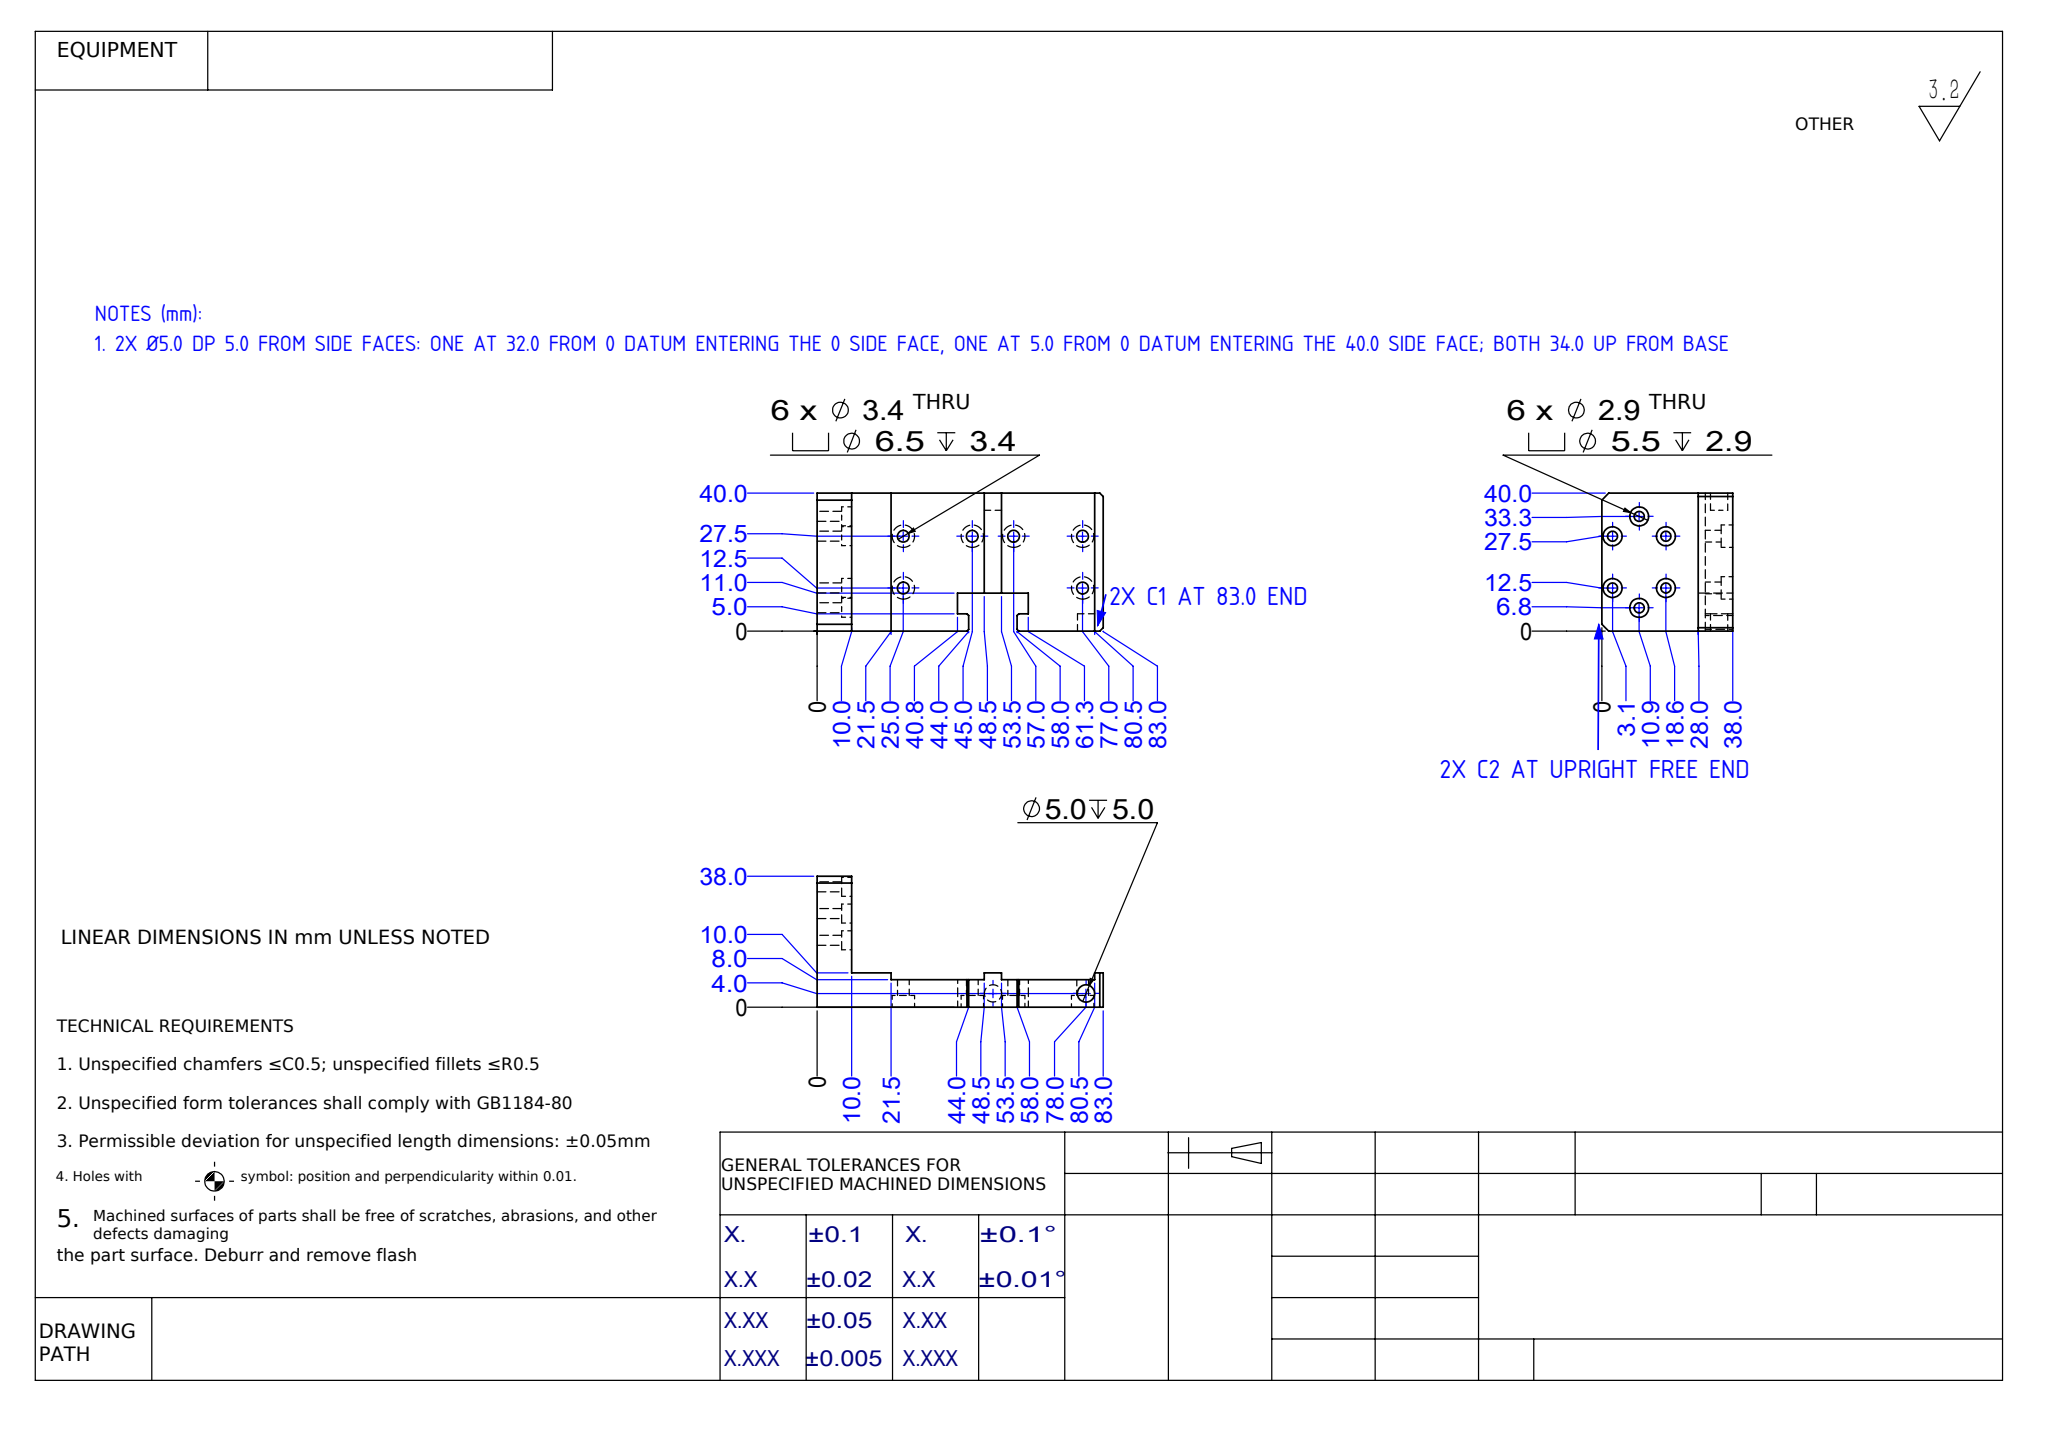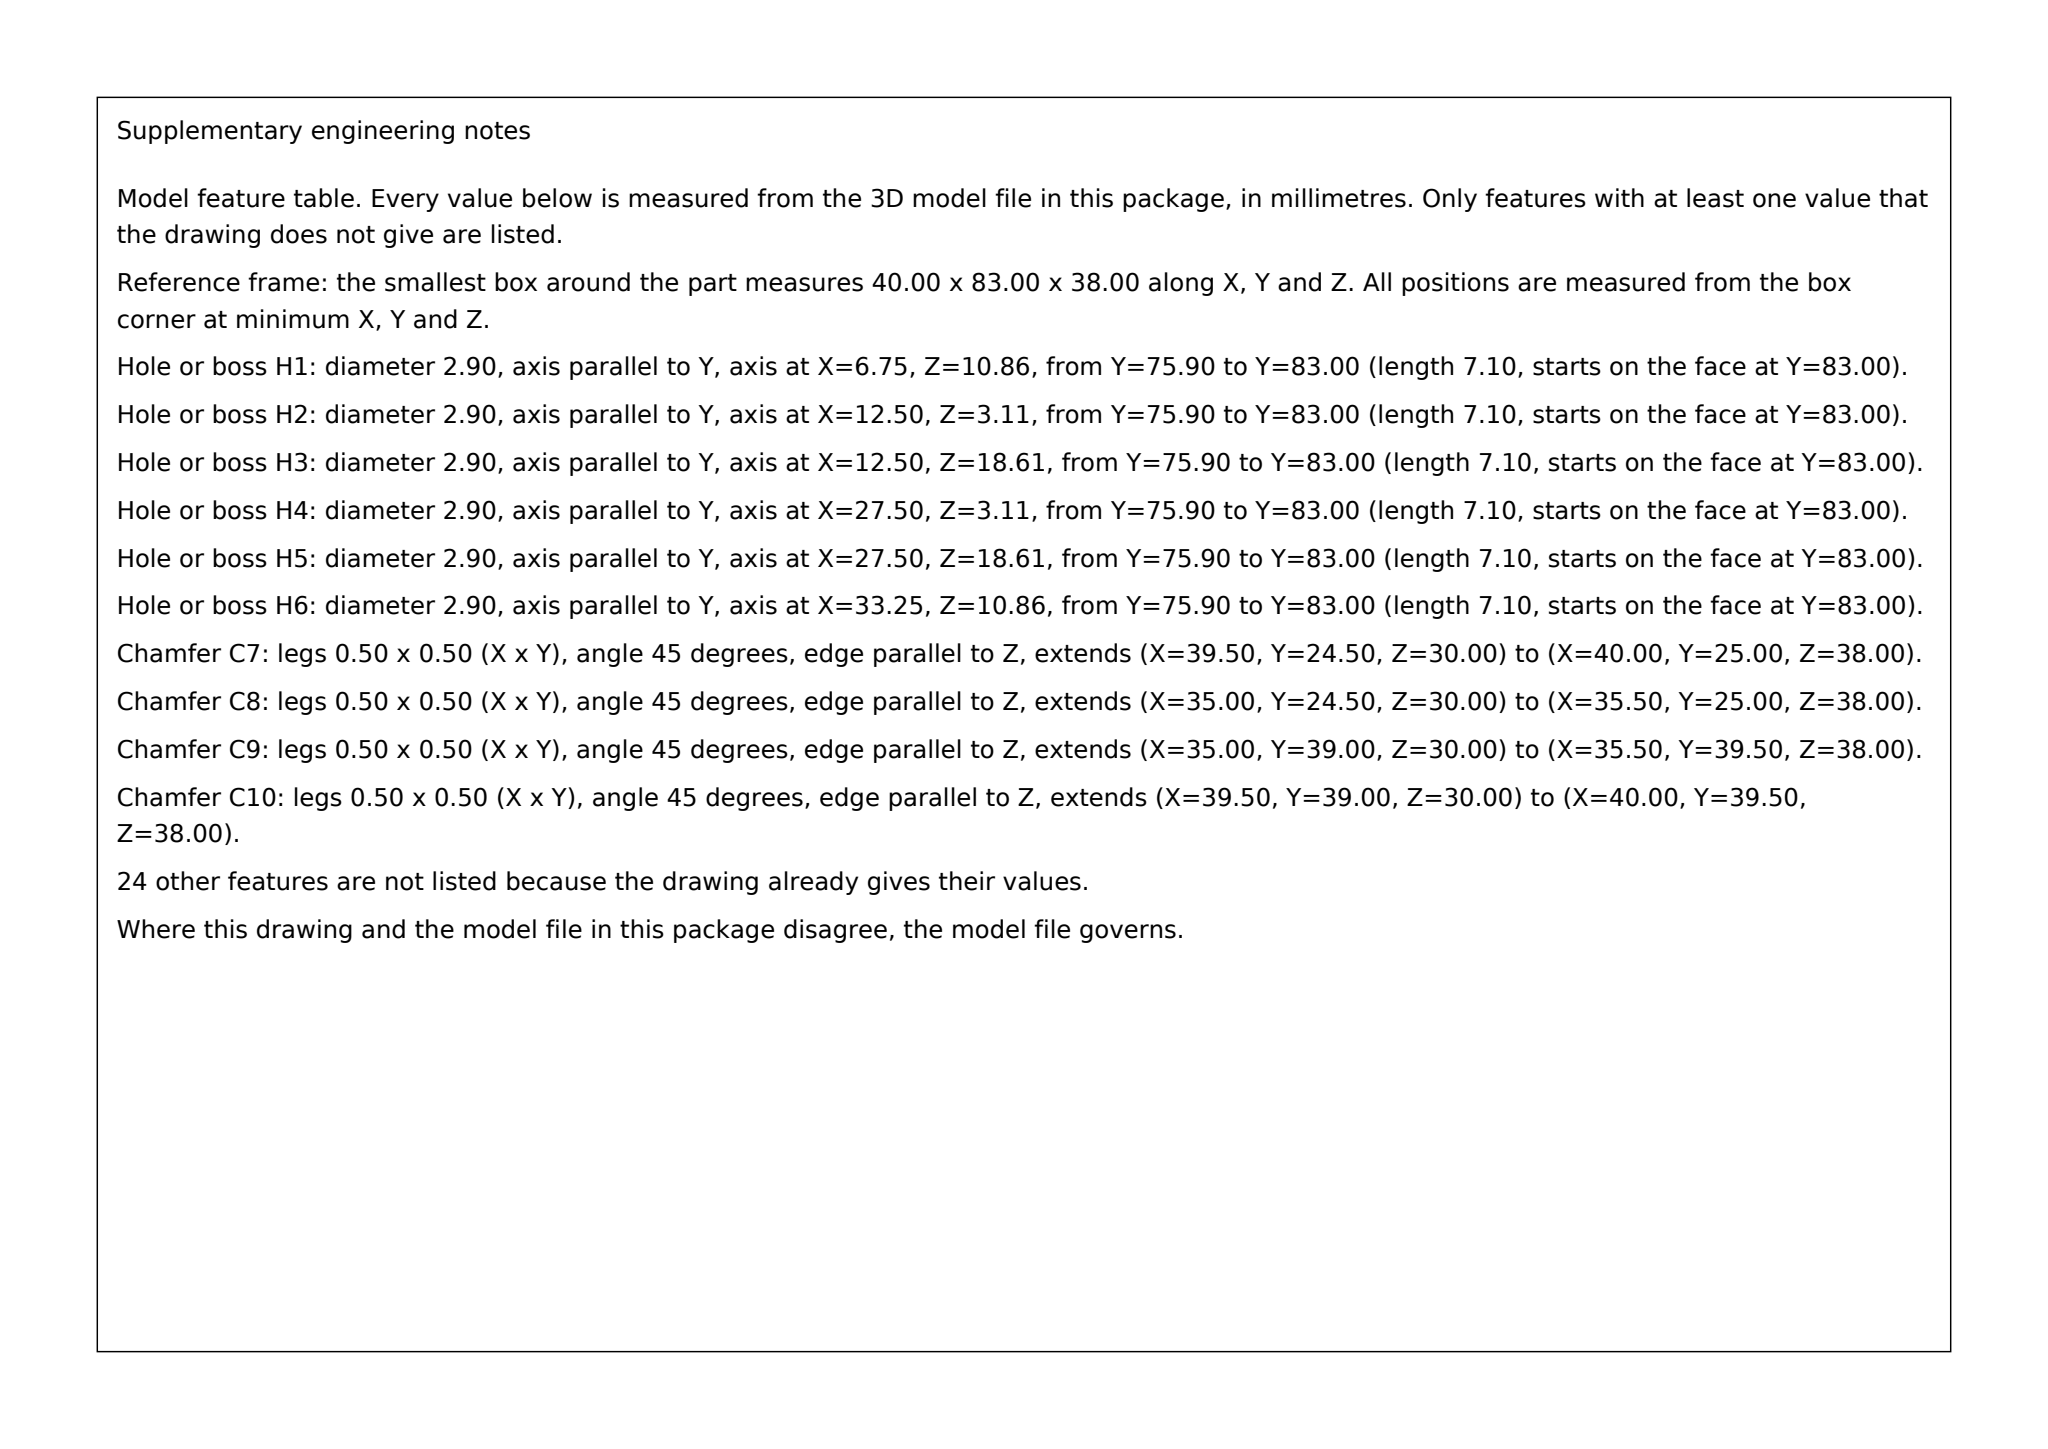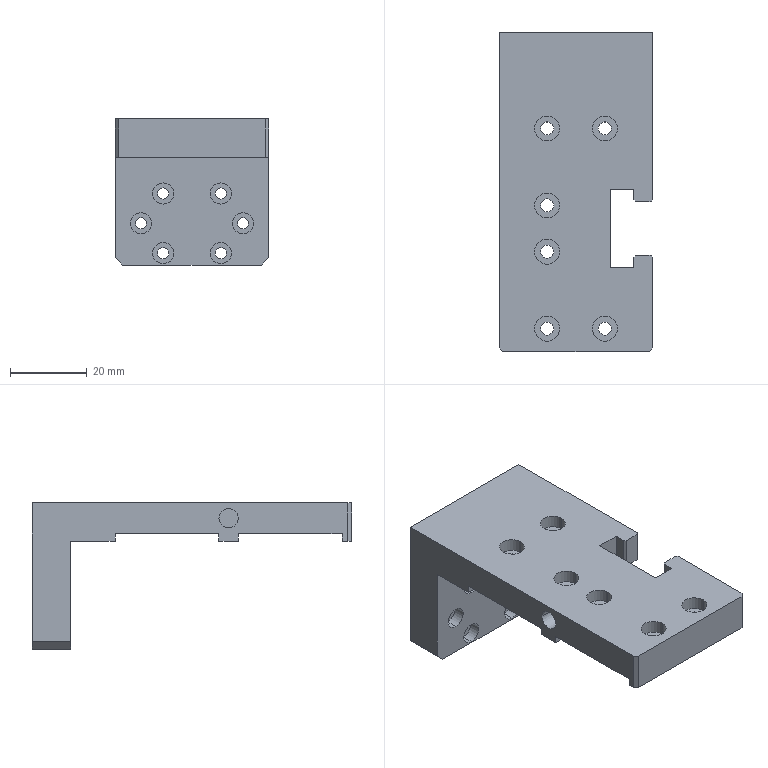Part | SolidWorks | mm | 1 solid | 98 faces | box 40 x 83 x 38 mm | volume 36553 mm3 | cylinder 52 | plane 46 | commonest cylinder face diameters 6.5 x12 3.4 x12 5.5 x12 2.9 x12 5 x4
Drawing notes:
2X Ø5.0 DP 5.0 FROM SIDE FACES: ONE AT 32.0 FROM 0 DATUM ENTERING THE 0 SIDE FACE, ONE AT 5.0 FROM 0 DATUM ENTERING THE 40.0 SIDE FACE; BOTH 34.0 UP FROM BASE | from the solid: cylinders: ["hole/bore",5.0,"x",[null,32.0,34.0],from 0.0 to 5.0] and ["hole/bore",5.0,"x",[null,5.0,34.0],from 35.0 to 40.0]; bbox_xyz [40.0,83.0,38.0]
2 X C2 ON UPRIGHT FREE-END VERT CORNERS (0 & 40.0 SIDES), 10 LG | from the solid: inclined_planes 45/45/90 at bbox_from [0,73,0] and [38,73,0], size [2,10,2] -> 2x2 chamfer on x=0 and x=40 corners of z=0 wall edge, 10 long in y (73-83)
2 X C1 ON 83.0 END CORNERS OF PLATE, FULL 10 PLATE HT | from the solid: inclined_planes 45/45/90 at bbox_from [0,0,28] and [39,0,28], size [1,1,10] -> 1x1 chamfer on x=0 and x=40 corners of plate free end (drawing 83.0), through z 28-38 (10 thk)
build123d program:
from build123d import *

# Parameters (mm, degrees)
SKETCH2_W                                         = 40
SKETCH2_H                                         = 73
BOSS_EXTRUDE2_DEPTH                               = 10
SKETCH3_W                                         = 40
SKETCH3_H                                         = 38
BOSS_EXTRUDE3_DEPTH                               = 10
M2_5_HEX_SOCKET_HEAD_CAP_SCREW_CBORE1_D           = 2.9
M2_5_HEX_SOCKET_HEAD_CAP_SCREW_CBORE1_CBORE_D     = 5.5
M2_5_HEX_SOCKET_HEAD_CAP_SCREW_CBORE1_CBORE_DEPTH = 2.9
SKETCH6_W                                         = 5
SKETCH6_H                                         = 14
CUT_EXTRUDE1_DEPTH                                = 64.295
SKETCH7_W                                         = 6
SKETCH7_H                                         = 20.5
CUT_EXTRUDE2_DEPTH                                = 64.295
M3_HEX_SOCKET_HEAD_CAP_SCREW_CBORE1_D             = 3.4
M3_HEX_SOCKET_HEAD_CAP_SCREW_CBORE1_CBORE_D       = 6.5
M3_HEX_SOCKET_HEAD_CAP_SCREW_CBORE1_CBORE_DEPTH   = 3.4
SKETCH10_W                                        = 40
SKETCH10_H                                        = 27
CUT_EXTRUDE3_DEPTH                                = 2
CHAMFER1_SIZE                                     = 2
CHAMFER2_SIZE                                     = 1
CHAMFER3_SIZE                                     = 0.5
SKETCH11_R                                        = 2.5
CUT_EXTRUDE4_DEPTH                                = 5
SKETCH12_R                                        = 2.5
CUT_EXTRUDE5_DEPTH                                = 5


with BuildPart() as part:
    # Sketch2 → Boss-Extrude2 (new body)
    with BuildSketch(Plane.XY):
        Rectangle(SKETCH2_W, SKETCH2_H)
    extrude(amount=BOSS_EXTRUDE2_DEPTH)

    # Sketch3 → Boss-Extrude3 (add)
    with BuildSketch(Plane(origin=(0, 36.5, 0), x_dir=(1, 0, 0), z_dir=(0, 1, 0))):
        with Locations((0, 9)):
            Rectangle(SKETCH3_W, SKETCH3_H)
    extrude(amount=BOSS_EXTRUDE3_DEPTH)

    # M2.5 Hex Socket Head Cap Screw CBORE1 (through all)
    with Locations(Plane(origin=(0, 36.5, 0), x_dir=(-1, 0, 0), z_dir=(0, -1, 0))):
        with Locations((-7.5, 9.385), (-13.25, 17.135), (-7.5, 24.885), (7.5, 24.885), (13.25, 17.135), (7.5, 9.385)):
            CounterBoreHole(M2_5_HEX_SOCKET_HEAD_CAP_SCREW_CBORE1_D / 2, M2_5_HEX_SOCKET_HEAD_CAP_SCREW_CBORE1_CBORE_D / 2, M2_5_HEX_SOCKET_HEAD_CAP_SCREW_CBORE1_CBORE_DEPTH)

    # Sketch6 → Cut-Extrude1 (cut, through all)
    with BuildSketch(Plane.XY.offset(10)):
        with Locations((17.5, -4.5)):
            Rectangle(SKETCH6_W, SKETCH6_H)
    extrude(amount=-CUT_EXTRUDE1_DEPTH, mode=Mode.SUBTRACT)

    # Sketch7 → Cut-Extrude2 (cut, through all)
    with BuildSketch(Plane.XY.offset(10)):
        with Locations((12, -4.5)):
            Rectangle(SKETCH7_W, SKETCH7_H)
    extrude(amount=-CUT_EXTRUDE2_DEPTH, mode=Mode.SUBTRACT)

    # M3 Hex Socket Head Cap Screw CBORE1 (through all)
    with Locations(Plane.XY.offset(10)):
        with Locations((-7.5, 1.5), (-7.5, 21.5), (7.5, 21.5), (-7.5, -10.5), (-7.5, -30.5), (7.5, -30.5)):
            CounterBoreHole(M3_HEX_SOCKET_HEAD_CAP_SCREW_CBORE1_D / 2, M3_HEX_SOCKET_HEAD_CAP_SCREW_CBORE1_CBORE_D / 2, M3_HEX_SOCKET_HEAD_CAP_SCREW_CBORE1_CBORE_DEPTH)

    # Sketch10 → Cut-Extrude3 (cut)
    with BuildSketch(Plane(origin=(0, 0, 0), x_dir=(-1, 0, 0), z_dir=(0, 0, -1))):
        with Locations((0, -20.5)):
            Rectangle(SKETCH10_W, SKETCH10_H)
        with Locations((0, 11.5)):
            Rectangle(SKETCH10_W, SKETCH10_H)
    extrude(amount=-CUT_EXTRUDE3_DEPTH, mode=Mode.SUBTRACT)

    # Chamfer1
    chamfer1_edges = [part.edges().sort_by_distance(p)[0] for p in [
        (-20, 41.5, -28),
        (20, 41.5, -28),
    ]]
    chamfer(chamfer1_edges, length=CHAMFER1_SIZE)

    # Chamfer2
    chamfer2_edges = [part.edges().sort_by_distance(p)[0] for p in [
        (20, -36.5, 5),
        (-20, -36.5, 5),
    ]]
    chamfer(chamfer2_edges, length=CHAMFER2_SIZE)

    # Chamfer3
    chamfer3_edges = [part.edges().sort_by_distance(p)[0] for p in [
        (15, 2.5, 6),
        (15, -11.5, 6),
        (20, 2.5, 6),
        (20, -11.5, 6),
    ]]
    chamfer(chamfer3_edges, length=CHAMFER3_SIZE)

    # Sketch11 → Cut-Extrude4 (cut)
    with BuildSketch(Plane(origin=(20, 0, 0), x_dir=(0, 0, -1), z_dir=(1, 0, 0))):
        with Locations(Location((-6, -31.5, 0), (0, 0, 90))):
            Circle(SKETCH11_R)
    extrude(amount=-CUT_EXTRUDE4_DEPTH, mode=Mode.SUBTRACT)

    # Sketch12 → Cut-Extrude5 (cut)
    with BuildSketch(Plane.ZY.offset(20)):
        with Locations(Location((6, -4.5, 0), (0, 0, 270))):
            Circle(SKETCH12_R)
    extrude(amount=-CUT_EXTRUDE5_DEPTH, mode=Mode.SUBTRACT)


solid = part.part